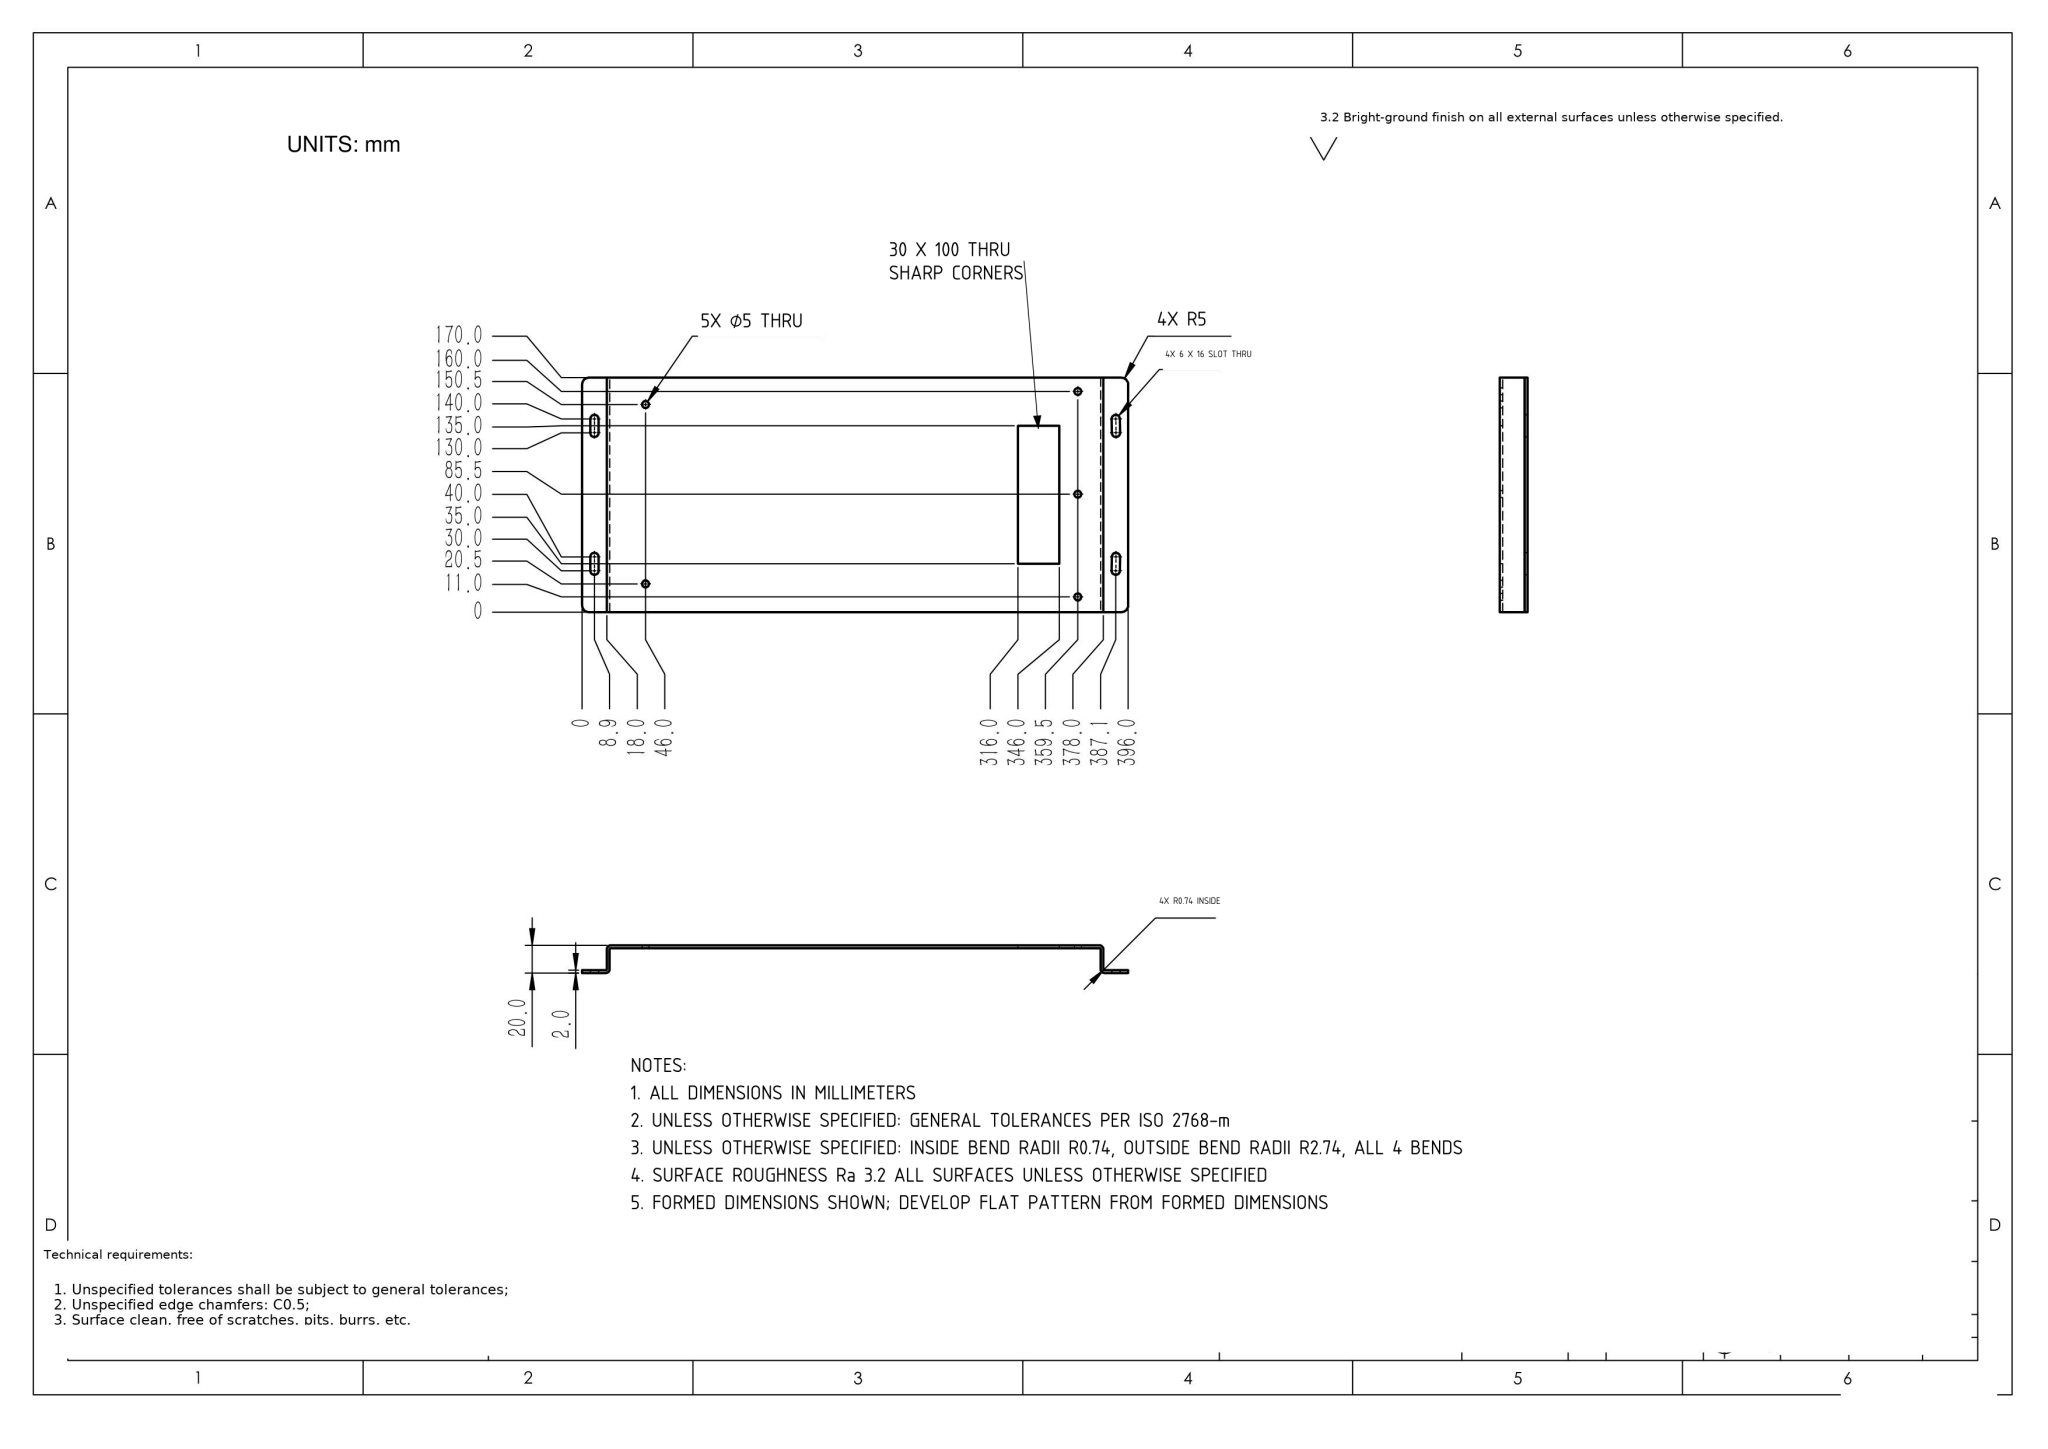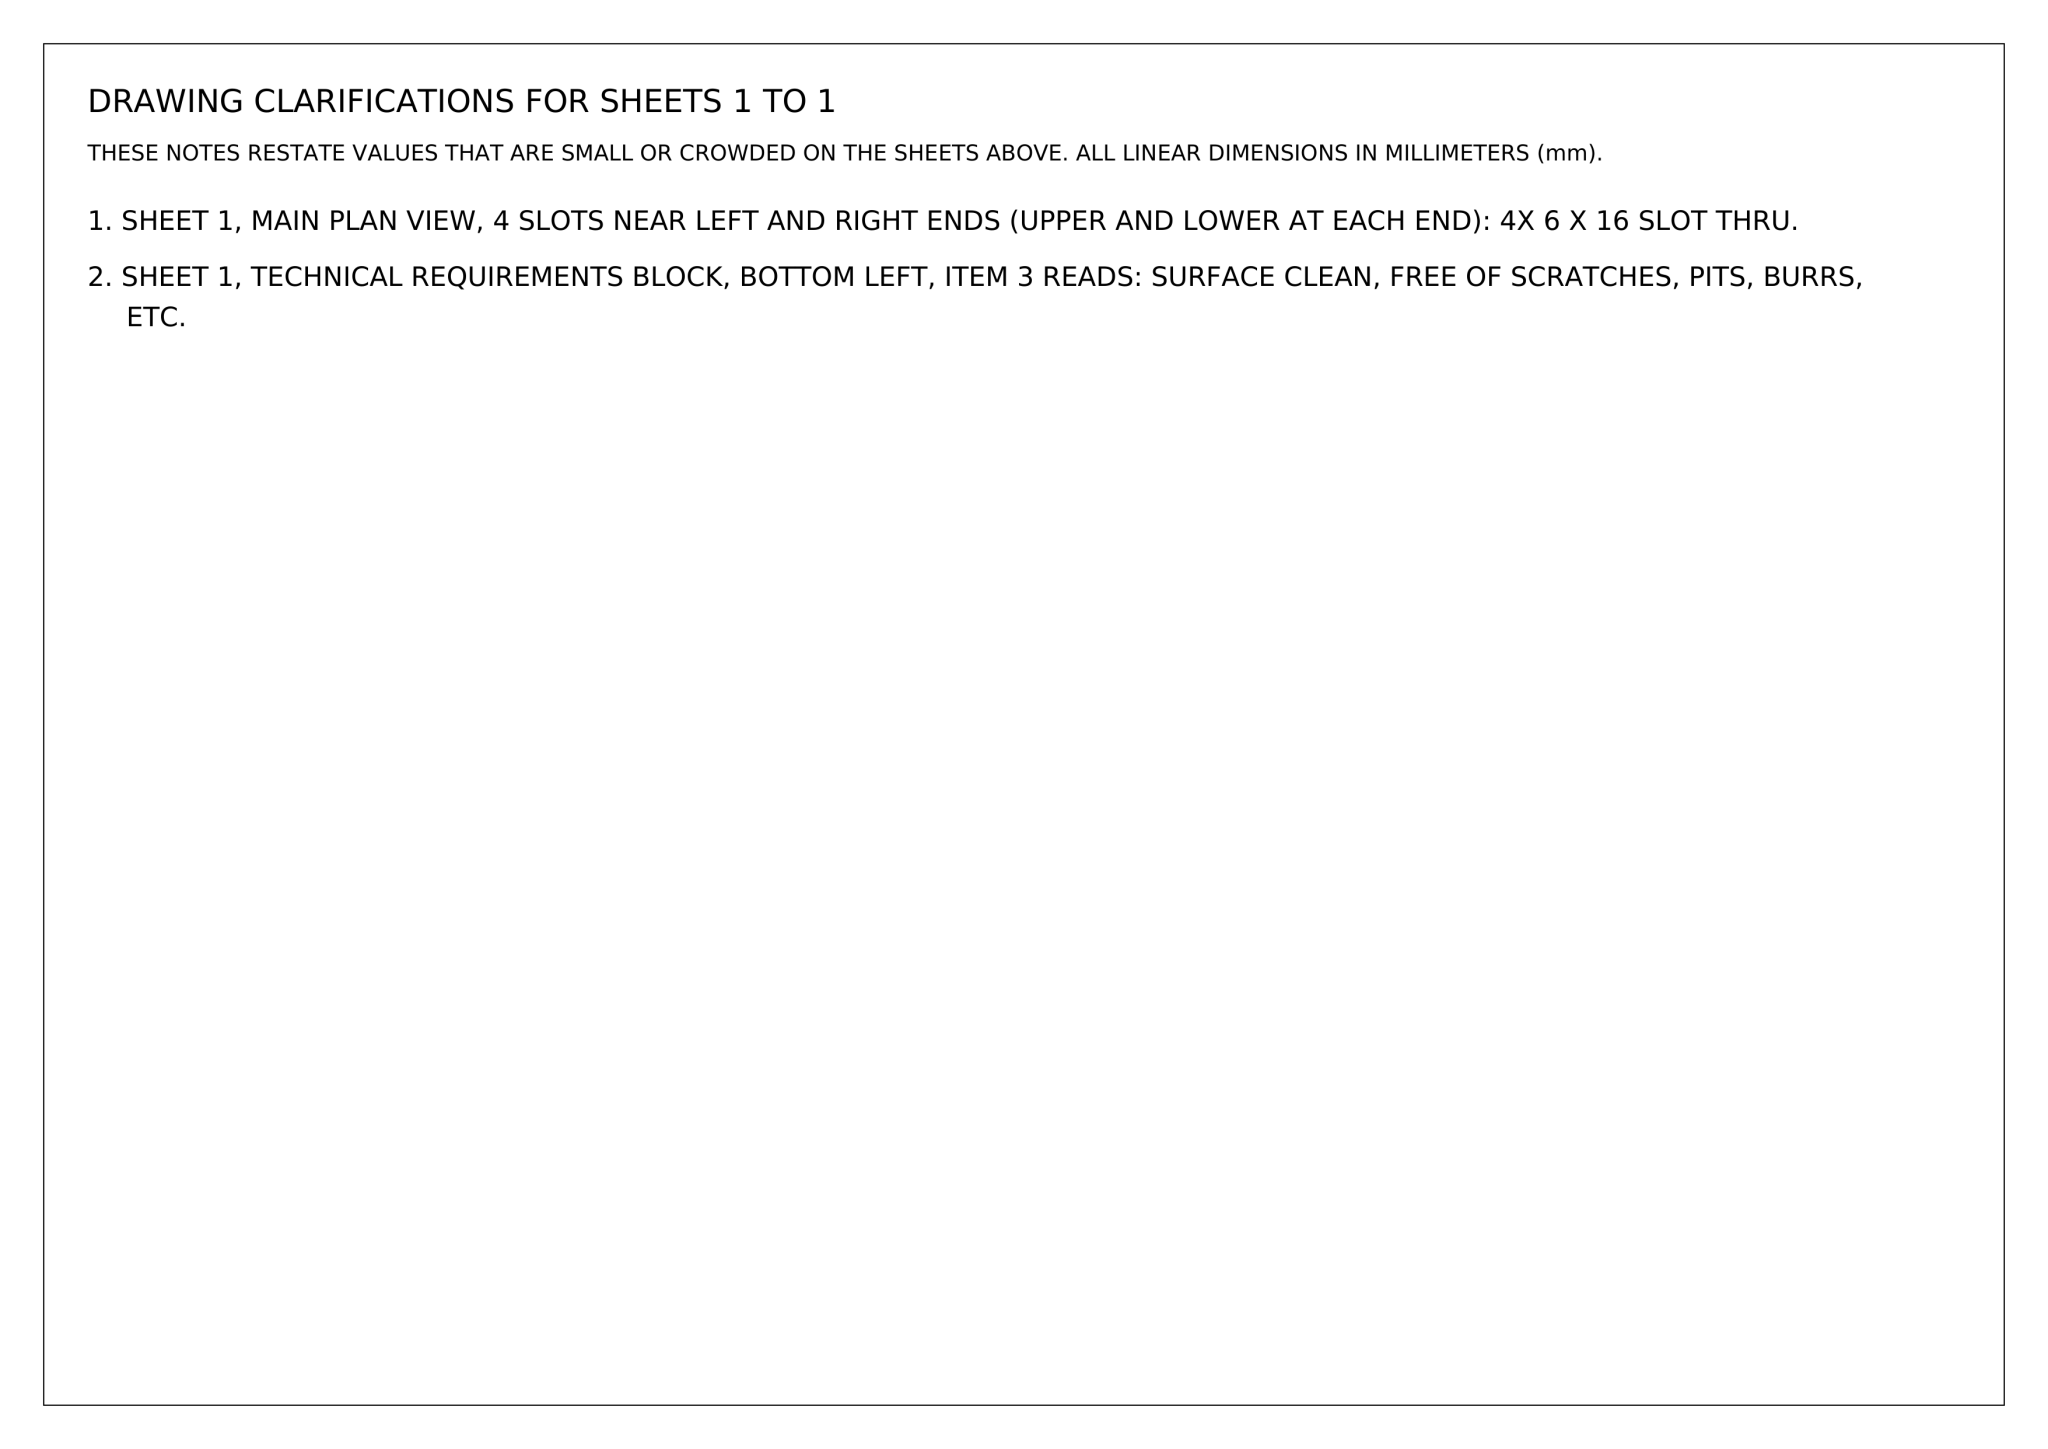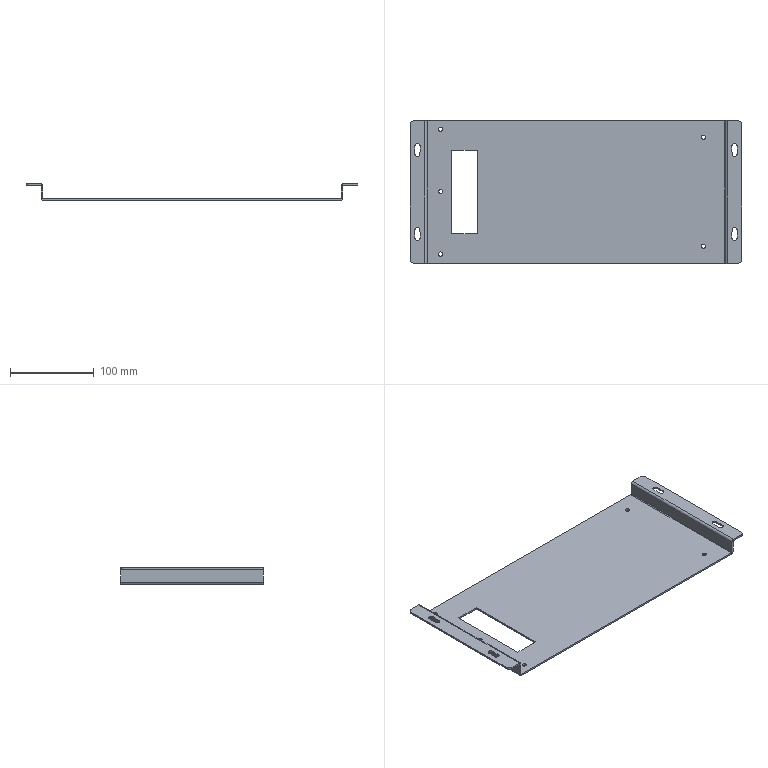Part | NX | mm | 1 solid | 76 faces | box 396 x 170 x 20 mm | volume 138921 mm3 | plane 42 | cylinder 34 | commonest cylinder face diameters 6 x12 5 x10 5.473 x4 1.473 x4 10 x4